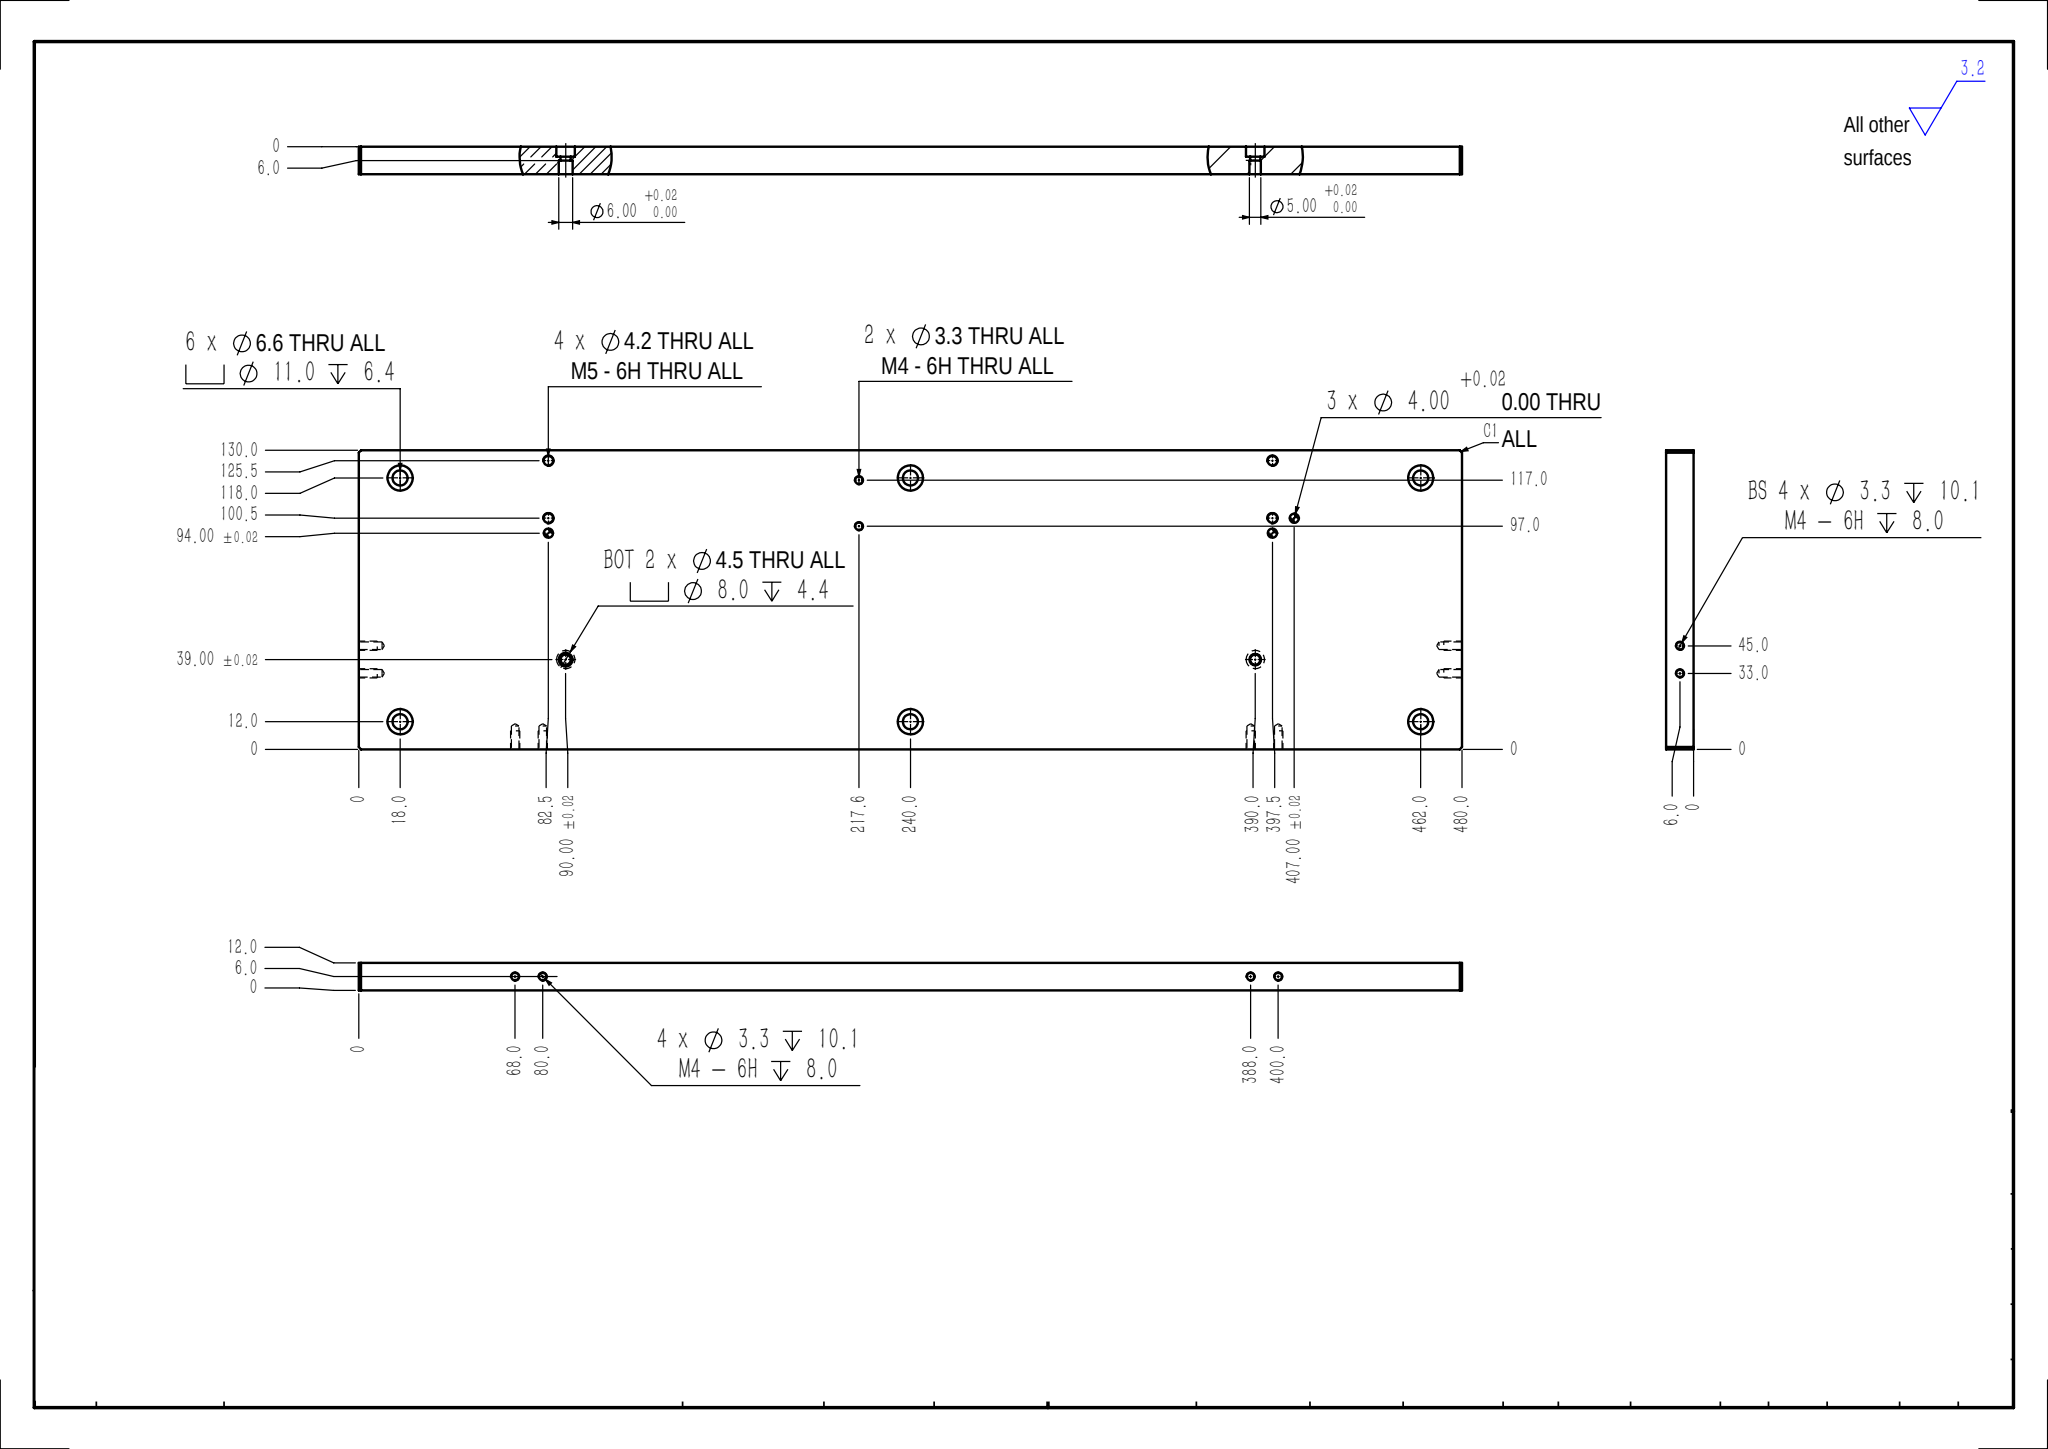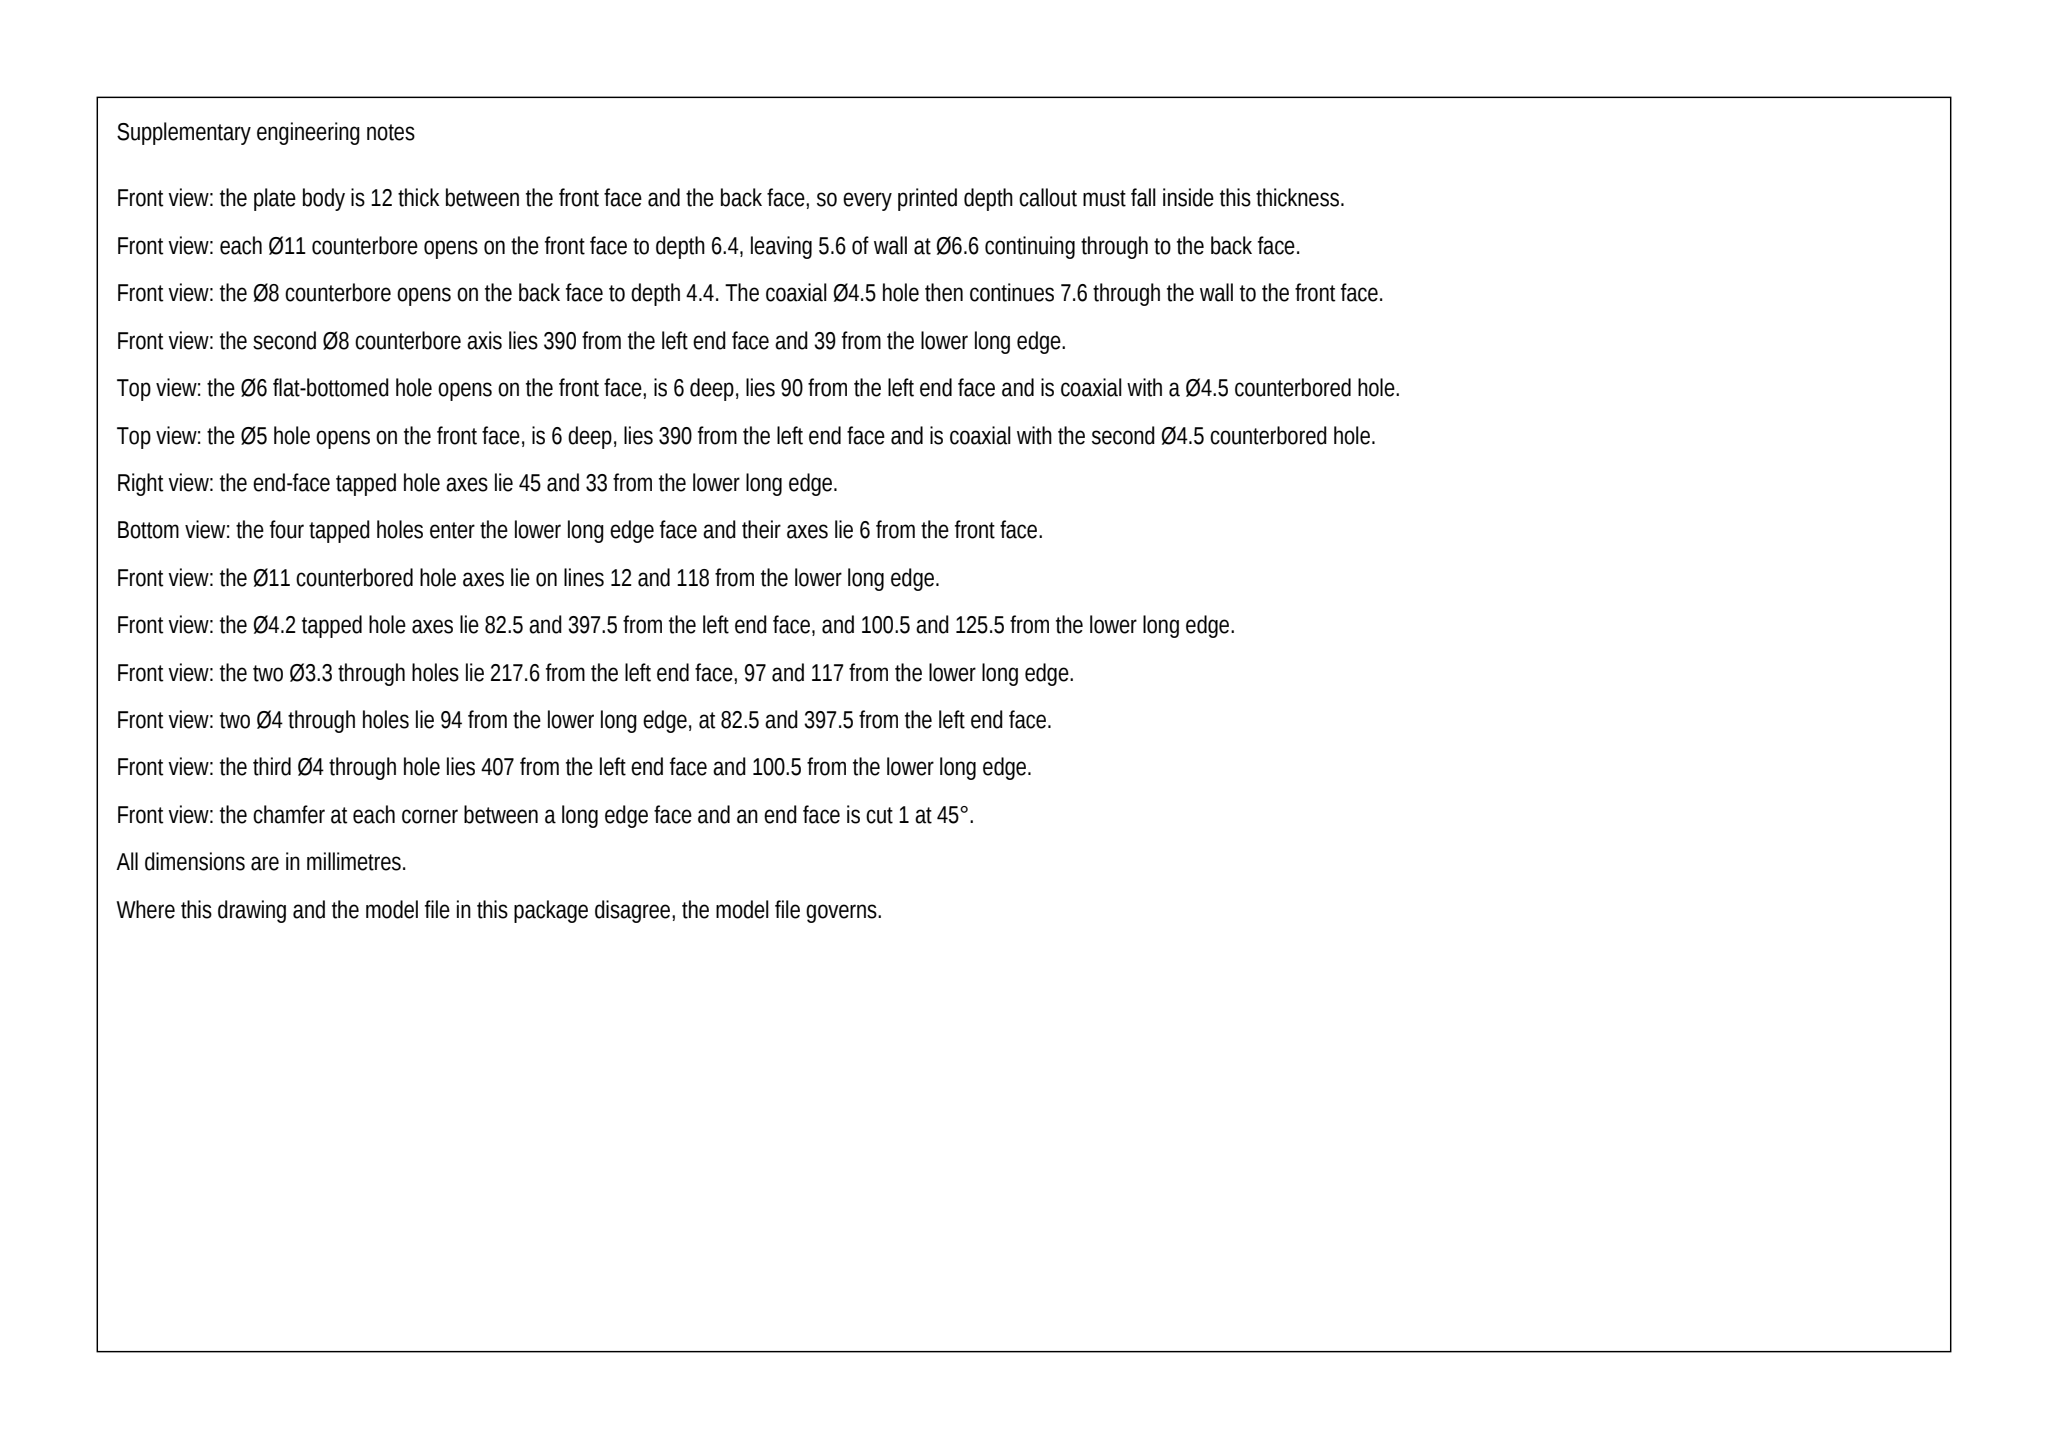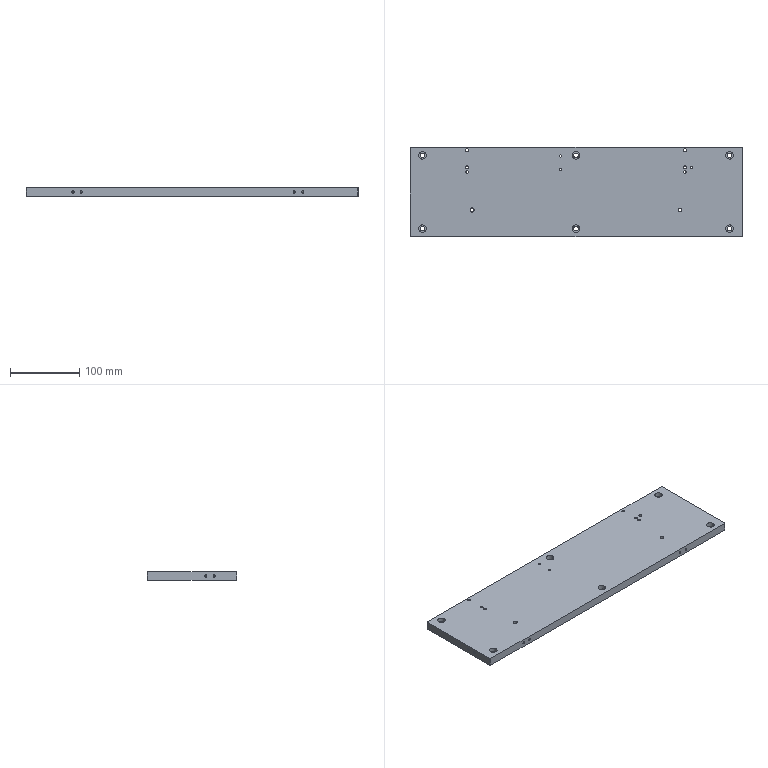Part | SolidWorks | mm | 1 solid | 106 faces | box 480 x 130 x 12 mm | volume 741160 mm3 | cylinder 70 | plane 20 | cone 16 | commonest cylinder face diameters 3.3 x20 11 x12 6.6 x12 4.2 x8 4 x6 8 x4 4.5 x4 5 x2
Drawing notes:
3 X Ø4.00 +0.02/0 THRU ALL | from the solid: Ø4.0 z-axis holes at (82.5,94.0), (397.5,94.0), (407.0,100.5), length 12.0 = full plate thickness
build123d program:
from build123d import *

# Parameters (mm, degrees)
SKETCH1_W                                       = 480
SKETCH1_H                                       = 130
BOSS_EXTRUDE1_DEPTH                             = 6
M6_HEX_SOCKET_HEAD_CAP_SCREW_CBORE1_D           = 6.6
M6_HEX_SOCKET_HEAD_CAP_SCREW_CBORE1_CBORE_D     = 11
M6_HEX_SOCKET_HEAD_CAP_SCREW_CBORE1_CBORE_DEPTH = 6.4
CHAMFER1_SIZE                                   = 1
M4_TAPPED_HOLE1_D                               = 3.3
M5_TAPPED_HOLE1_D                               = 4.2
SIZE_MM_DOWEL_HOLE1_D                           = 4
SIZE_MM_DOWEL_HOLE3_D                           = 6
SIZE_MM_DOWEL_HOLE3_DEPTH                       = 6
SIZE_MM_DOWEL_HOLE3_2_D                         = 5
SIZE_MM_DOWEL_HOLE3_2_DEPTH                     = 6
M4_HEX_SOCKET_HEAD_CAP_SCREW_CBORE1_D           = 4.5
M4_HEX_SOCKET_HEAD_CAP_SCREW_CBORE1_CBORE_D     = 8
M4_HEX_SOCKET_HEAD_CAP_SCREW_CBORE1_CBORE_DEPTH = 4.4
M4_TAPPED_HOLE2_D                               = 3.3
M4_TAPPED_HOLE2_DEPTH                           = 10.1
M4_TAPPED_HOLE2_TIP                             = 0.9914
M4_TAPPED_HOLE3_D                               = 3.3
M4_TAPPED_HOLE3_DEPTH                           = 10.1
M4_TAPPED_HOLE3_TIP                             = 0.9914
M4_TAPPED_HOLE4_D                               = 3.3
M4_TAPPED_HOLE4_DEPTH                           = 10.1
M4_TAPPED_HOLE4_TIP                             = 0.9914


with BuildPart() as part:
    # Sketch1 → Boss-Extrude1 (new, symmetric)
    with BuildSketch(Plane.XY):
        Rectangle(SKETCH1_W, SKETCH1_H)
    extrude(amount=BOSS_EXTRUDE1_DEPTH, both=True)

    # M6 Hex Socket Head Cap Screw CBORE1 (through all)
    with Locations(Plane.XY.offset(6)):
        with Locations((-222, 53), (0, 53), (-222, -53), (0, -53), (222, -53), (222, 53)):
            CounterBoreHole(M6_HEX_SOCKET_HEAD_CAP_SCREW_CBORE1_D / 2, M6_HEX_SOCKET_HEAD_CAP_SCREW_CBORE1_CBORE_D / 2, M6_HEX_SOCKET_HEAD_CAP_SCREW_CBORE1_CBORE_DEPTH)

    # Chamfer1
    chamfer1_edges = [part.edges().sort_by_distance(p)[0] for p in [
        (240, -65, 0),
        (-240, -65, 0),
        (-240, 65, 0),
        (240, 65, 0),
    ]]
    chamfer(chamfer1_edges, length=CHAMFER1_SIZE)

    # M4 Tapped Hole1 (through all)
    with Locations(Plane.XY.offset(6)):
        with Locations((-22.4, 32), (-22.4, 52)):
            Hole(M4_TAPPED_HOLE1_D / 2)

    # M5 Tapped Hole1 (through all)
    with Locations(Plane.XY.offset(6)):
        with Locations((157.5, 35.5), (157.5, 60.5), (-157.5, 35.5), (-157.5, 60.5)):
            Hole(M5_TAPPED_HOLE1_D / 2)

    # Size mm Dowel Hole1 (through all)
    with Locations(Plane.XY.offset(6)):
        with Locations((157.5, 29), (-157.5, 29), (167, 35.5)):
            Hole(SIZE_MM_DOWEL_HOLE1_D / 2)

    # Size mm Dowel Hole3
    with Locations(Plane.XY.offset(6)):
        with Locations((-150, -26)):
            Hole(SIZE_MM_DOWEL_HOLE3_D / 2, depth=SIZE_MM_DOWEL_HOLE3_DEPTH)

    # Size mm Dowel Hole3_2
    with Locations(Plane.XY.offset(6)):
        with Locations((150, -26)):
            Hole(SIZE_MM_DOWEL_HOLE3_2_D / 2, depth=SIZE_MM_DOWEL_HOLE3_2_DEPTH)

    # M4 Hex Socket Head Cap Screw CBORE1 (through all)
    with Locations(Plane(origin=(0, 0, -6), x_dir=(-1, 0, 0), z_dir=(0, 0, -1))):
        with Locations((150, -26), (-150, -26)):
            CounterBoreHole(M4_HEX_SOCKET_HEAD_CAP_SCREW_CBORE1_D / 2, M4_HEX_SOCKET_HEAD_CAP_SCREW_CBORE1_CBORE_D / 2, M4_HEX_SOCKET_HEAD_CAP_SCREW_CBORE1_CBORE_DEPTH)

    # M4 Tapped Hole2
    with Locations(Plane.ZY.offset(240)):
        with Locations((0, -20), (0, -32)):
            Hole(M4_TAPPED_HOLE2_D / 2, depth=M4_TAPPED_HOLE2_DEPTH)
            with Locations((0, 0, -(M4_TAPPED_HOLE2_DEPTH + M4_TAPPED_HOLE2_TIP / 2))):  # 118° drill point
                Cone(0, M4_TAPPED_HOLE2_D / 2, M4_TAPPED_HOLE2_TIP, mode=Mode.SUBTRACT)

    # M4 Tapped Hole3
    with Locations(Plane(origin=(0, -65, 0), x_dir=(-1, 0, 0), z_dir=(0, -1, 0))):
        with Locations((172, 0), (160, 0), (-148, 0), (-160, 0)):
            Hole(M4_TAPPED_HOLE3_D / 2, depth=M4_TAPPED_HOLE3_DEPTH)
            with Locations((0, 0, -(M4_TAPPED_HOLE3_DEPTH + M4_TAPPED_HOLE3_TIP / 2))):  # 118° drill point
                Cone(0, M4_TAPPED_HOLE3_D / 2, M4_TAPPED_HOLE3_TIP, mode=Mode.SUBTRACT)

    # M4 Tapped Hole4
    with Locations(Plane(origin=(240, 0, 0), x_dir=(0, 0, -1), z_dir=(1, 0, 0))):
        with Locations((0, -32), (0, -20)):
            Hole(M4_TAPPED_HOLE4_D / 2, depth=M4_TAPPED_HOLE4_DEPTH)
            with Locations((0, 0, -(M4_TAPPED_HOLE4_DEPTH + M4_TAPPED_HOLE4_TIP / 2))):  # 118° drill point
                Cone(0, M4_TAPPED_HOLE4_D / 2, M4_TAPPED_HOLE4_TIP, mode=Mode.SUBTRACT)


solid = part.part